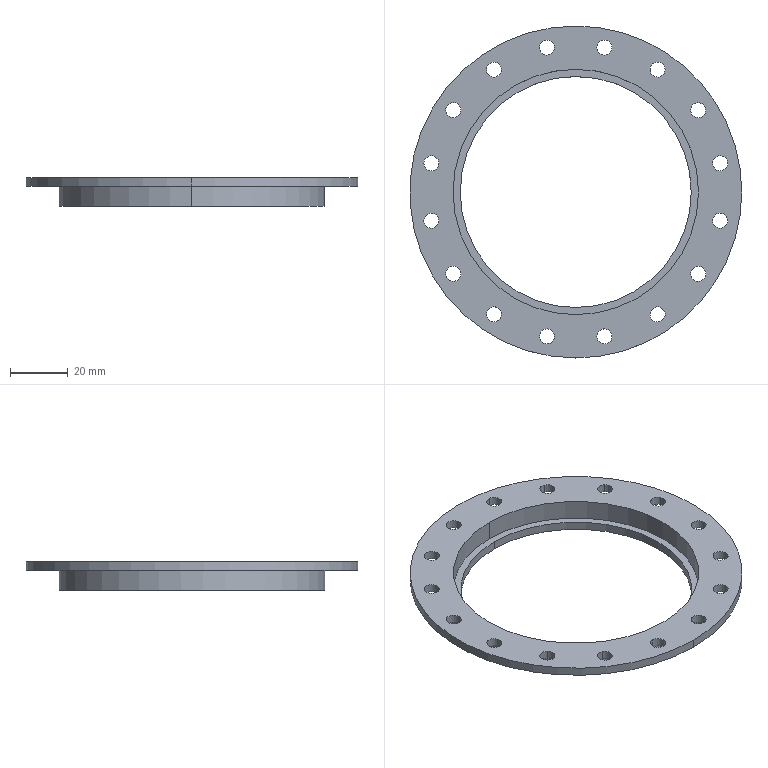CAM job | Mastercam | mm | 1 operations | part box 115 x 115 x 10
1. Drill/Counterbore | 5 - 4 倒角刀